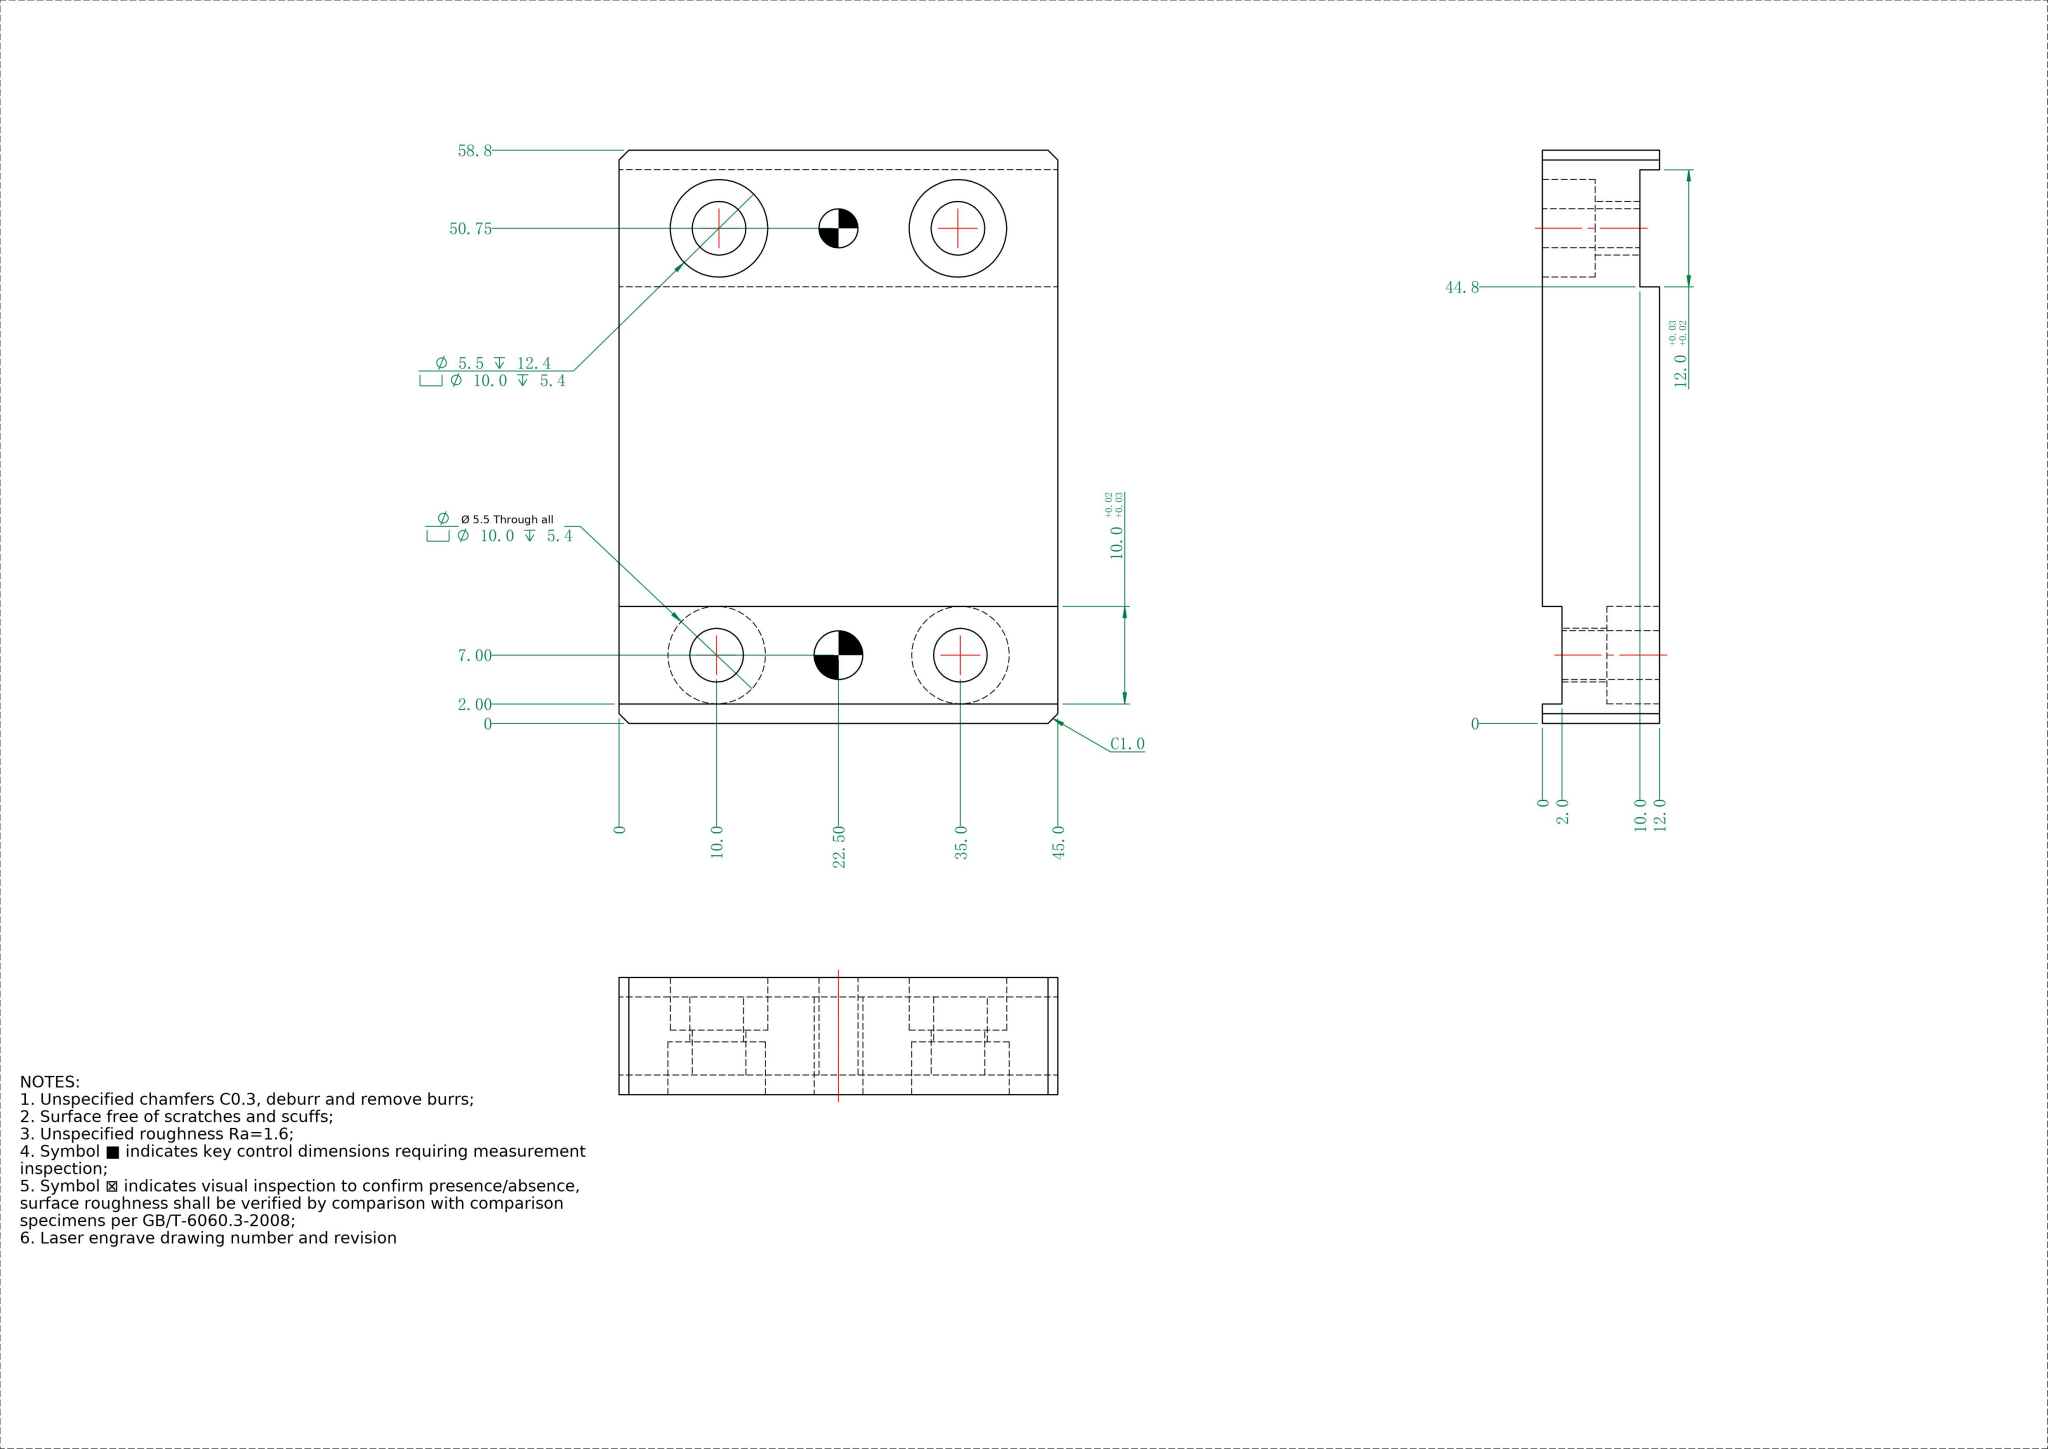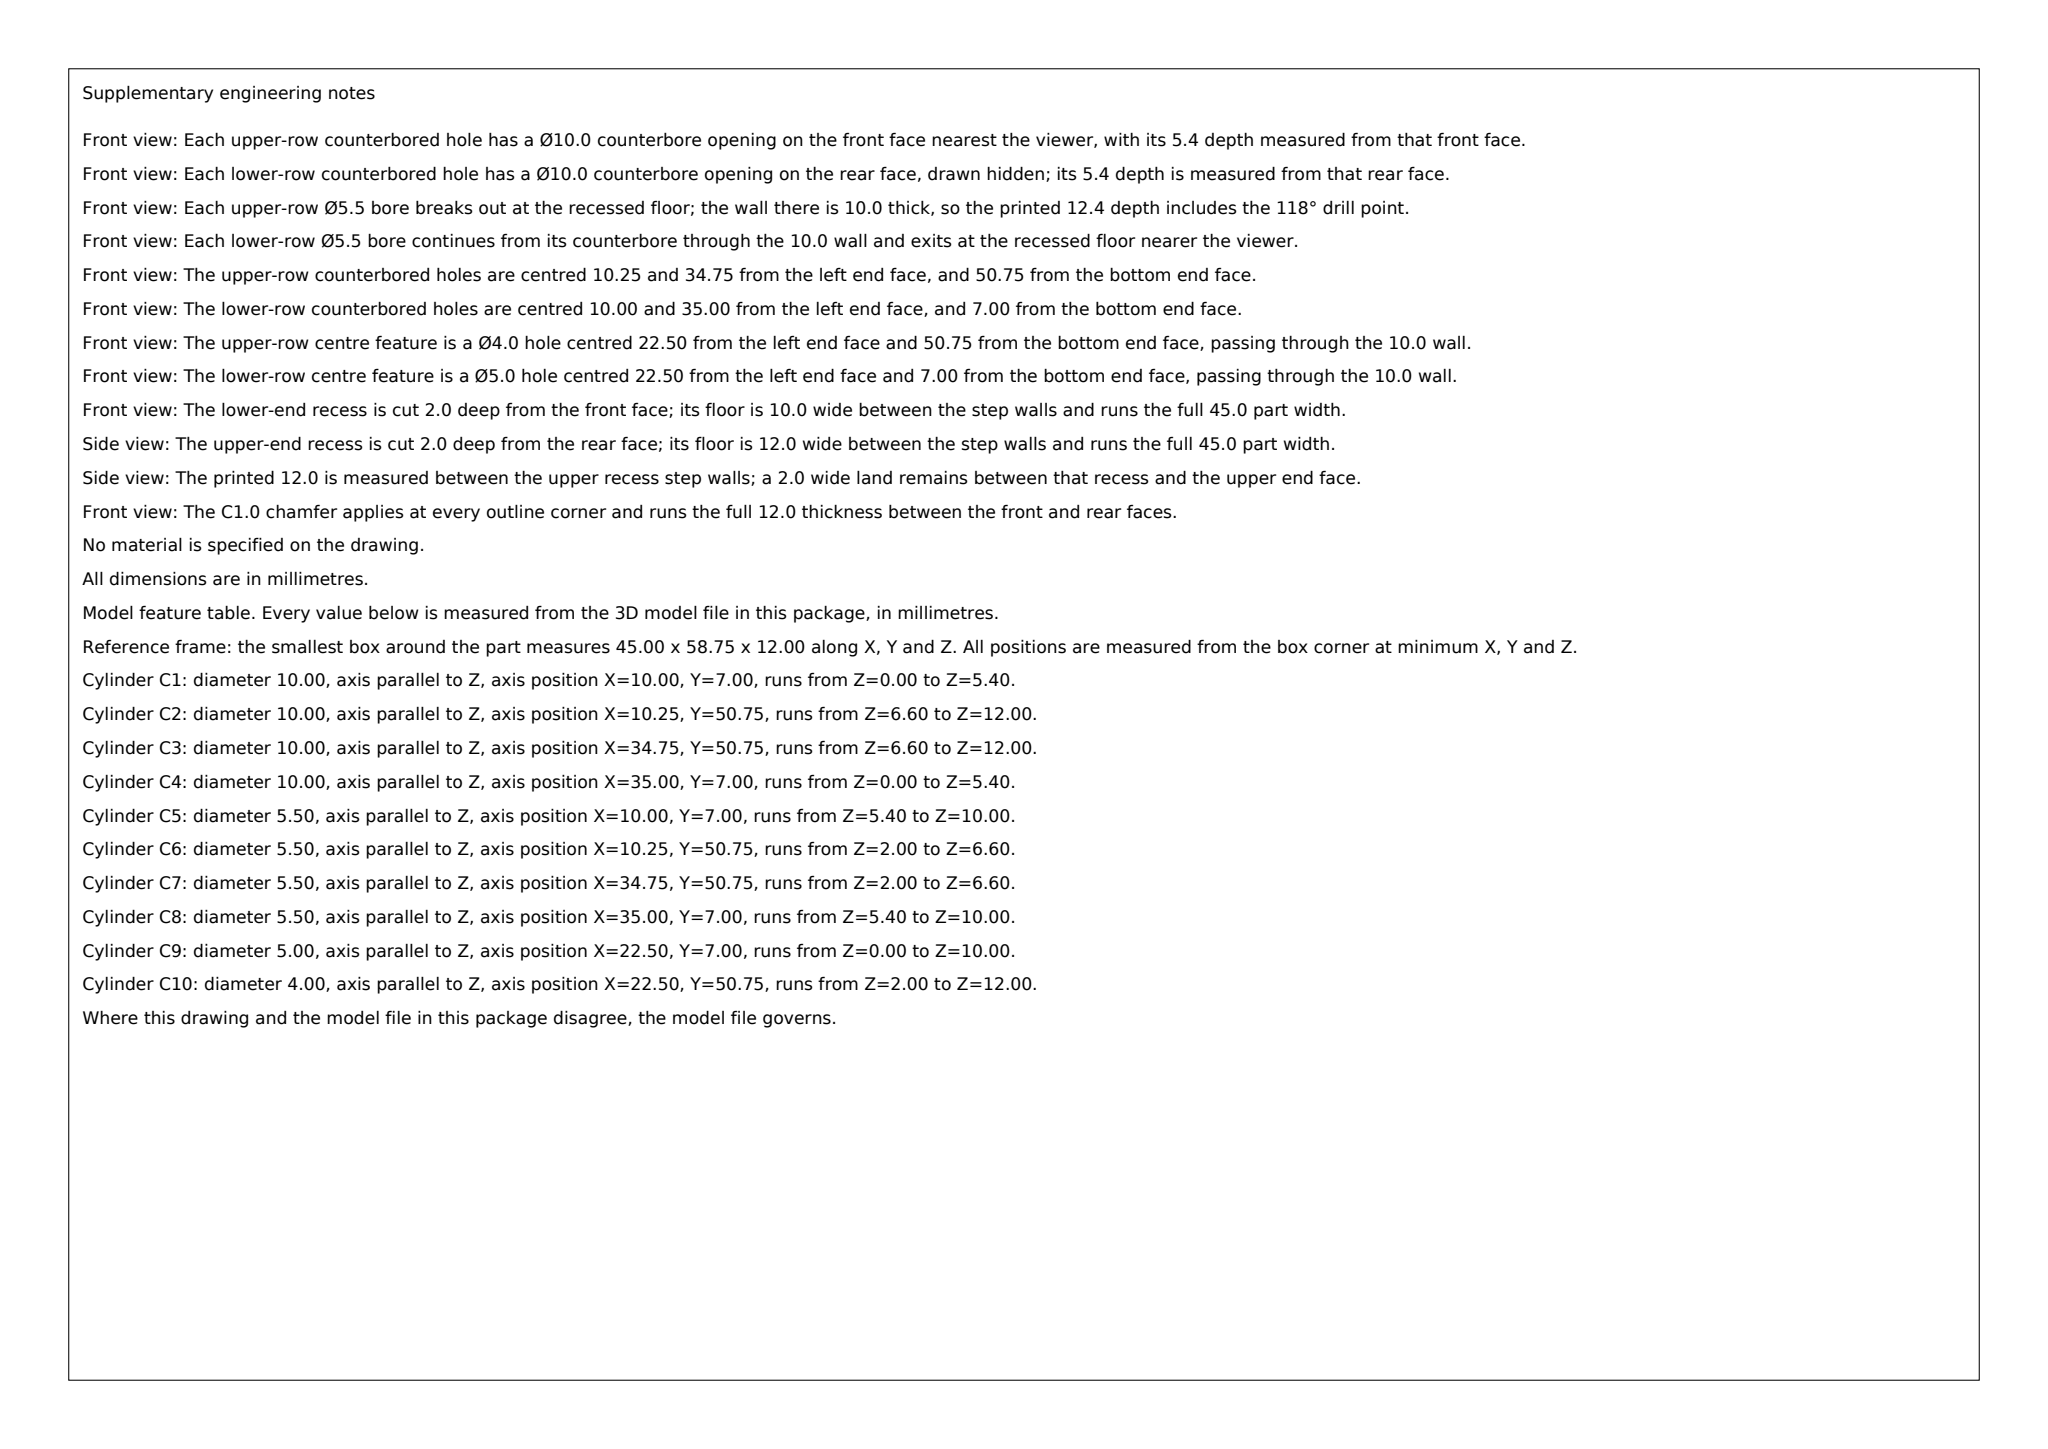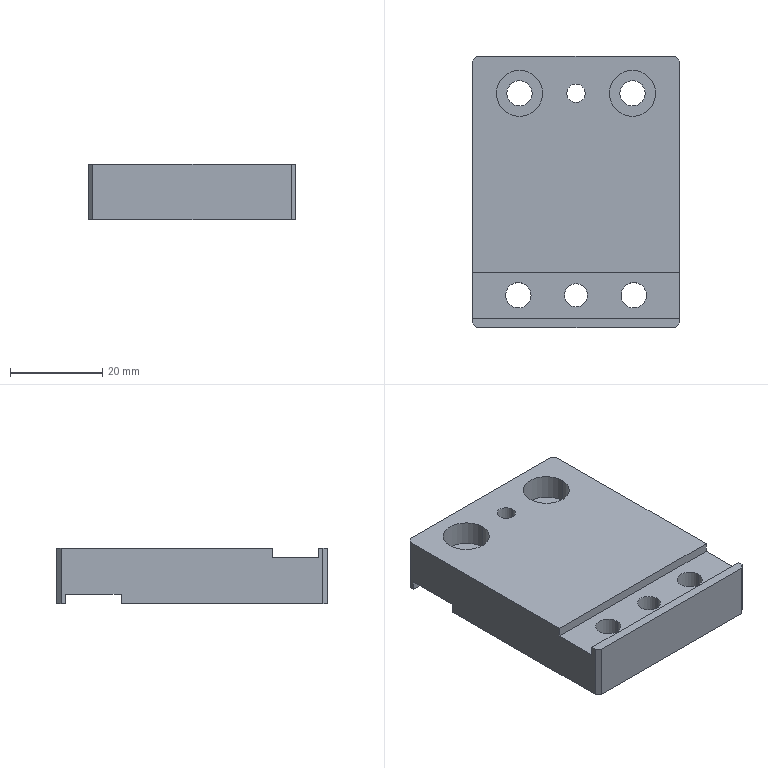Part | SolidWorks | mm | 1 solid | 42 faces | box 45 x 58.75 x 12 mm | volume 27265 mm3 | plane 22 | cylinder 20 | commonest cylinder face diameters 10 x8 5.5 x8 4 x2 5 x2
build123d program:
from build123d import *

# Parameters (mm, degrees)
SKETCH1_W                                       = 45
SKETCH1_H                                       = 58.75
BOSS_EXTRUDE1_DEPTH                             = 12
SKETCH2_W                                       = 2
SKETCH2_H                                       = 12
CUT_EXTRUDE1_DEPTH                              = 75.97
SKETCH3_W                                       = 2
SKETCH3_H                                       = 10
CUT_EXTRUDE2_DEPTH                              = 75.97
M5_HEX_SOCKET_HEAD_CAP_SCREW_CBORE1_D           = 5.5
M5_HEX_SOCKET_HEAD_CAP_SCREW_CBORE1_CBORE_D     = 10
M5_HEX_SOCKET_HEAD_CAP_SCREW_CBORE1_CBORE_DEPTH = 5.4
SIZE_MM_DOWEL_PIN_HOLE_1_D                      = 5
M5_HEX_SOCKET_HEAD_CAP_SCREW_CBORE2_D           = 5.5
M5_HEX_SOCKET_HEAD_CAP_SCREW_CBORE2_DEPTH       = 12.4
M5_HEX_SOCKET_HEAD_CAP_SCREW_CBORE2_CBORE_D     = 10
M5_HEX_SOCKET_HEAD_CAP_SCREW_CBORE2_CBORE_DEPTH = 5.4
M5_HEX_SOCKET_HEAD_CAP_SCREW_CBORE2_TIP         = 1.652
SIZE_MM_DOWEL_PIN_HOLE_2_D                      = 4
SIZE_MM_DOWEL_PIN_HOLE_2_DEPTH                  = 12.4
SIZE_MM_DOWEL_PIN_HOLE_2_TIP                    = 1.202
CHAMFER1_SIZE                                   = 1


with BuildPart() as part:
    # Sketch1 → Boss-Extrude1 (new body)
    with BuildSketch(Plane.XY):
        with Locations((22.5, 29.375)):
            Rectangle(SKETCH1_W, SKETCH1_H)
    extrude(amount=BOSS_EXTRUDE1_DEPTH)

    # Sketch2 → Cut-Extrude1 (cut, through all)
    with BuildSketch(Plane.ZY):
        with Locations((1, 50.75)):
            Rectangle(SKETCH2_W, SKETCH2_H)
    extrude(amount=-CUT_EXTRUDE1_DEPTH, mode=Mode.SUBTRACT)

    # Sketch3 → Cut-Extrude2 (cut, through all)
    with BuildSketch(Plane.ZY):
        with Locations((11, 7)):
            Rectangle(SKETCH3_W, SKETCH3_H)
    extrude(amount=-CUT_EXTRUDE2_DEPTH, mode=Mode.SUBTRACT)

    # M5 Hex Socket Head Cap Screw CBORE1 (through all)
    with Locations(Plane(origin=(0, 0, 0), x_dir=(-1, 0, 0), z_dir=(0, 0, -1))):
        with Locations((-35.003, 7), (-10.003, 7)):
            CounterBoreHole(M5_HEX_SOCKET_HEAD_CAP_SCREW_CBORE1_D / 2, M5_HEX_SOCKET_HEAD_CAP_SCREW_CBORE1_CBORE_D / 2, M5_HEX_SOCKET_HEAD_CAP_SCREW_CBORE1_CBORE_DEPTH)

    # Size mm Dowel Pin Hole 1 (through all)
    with Locations(Plane.XY.offset(10)):
        with Locations((22.503, 7)):
            Hole(SIZE_MM_DOWEL_PIN_HOLE_1_D / 2)

    # M5 Hex Socket Head Cap Screw CBORE2
    with Locations(Plane.XY.offset(12)):
        with Locations((34.75, 50.75), (10.25, 50.75)):
            CounterBoreHole(M5_HEX_SOCKET_HEAD_CAP_SCREW_CBORE2_D / 2, M5_HEX_SOCKET_HEAD_CAP_SCREW_CBORE2_CBORE_D / 2, M5_HEX_SOCKET_HEAD_CAP_SCREW_CBORE2_CBORE_DEPTH, depth=M5_HEX_SOCKET_HEAD_CAP_SCREW_CBORE2_DEPTH)
            with Locations((0, 0, -(M5_HEX_SOCKET_HEAD_CAP_SCREW_CBORE2_DEPTH + M5_HEX_SOCKET_HEAD_CAP_SCREW_CBORE2_TIP / 2))):  # 118° drill point
                Cone(0, M5_HEX_SOCKET_HEAD_CAP_SCREW_CBORE2_D / 2, M5_HEX_SOCKET_HEAD_CAP_SCREW_CBORE2_TIP, mode=Mode.SUBTRACT)

    # Size mm Dowel Pin Hole 2
    with Locations(Plane.XY.offset(12)):
        with Locations((22.5, 50.75)):
            Hole(SIZE_MM_DOWEL_PIN_HOLE_2_D / 2, depth=SIZE_MM_DOWEL_PIN_HOLE_2_DEPTH)
            with Locations((0, 0, -(SIZE_MM_DOWEL_PIN_HOLE_2_DEPTH + SIZE_MM_DOWEL_PIN_HOLE_2_TIP / 2))):  # 118° drill point
                Cone(0, SIZE_MM_DOWEL_PIN_HOLE_2_D / 2, SIZE_MM_DOWEL_PIN_HOLE_2_TIP, mode=Mode.SUBTRACT)

    # Chamfer1
    chamfer1_edges = [part.edges().sort_by_distance(p)[0] for p in [
        (0, 58.75, 6),
        (45, 58.75, 6),
        (45, 0, 6),
        (0, 0, 6),
    ]]
    chamfer(chamfer1_edges, length=CHAMFER1_SIZE)


solid = part.part